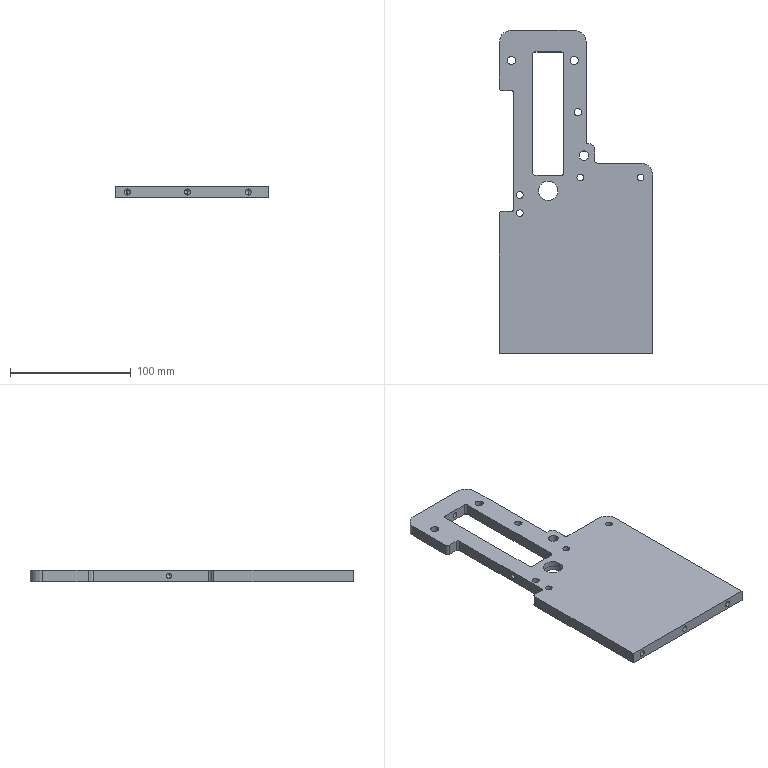Component | SolidWorks | FrameRightPlate.1-1 | 1 solid | 70 faces | box 127 x 268 x 9.4 mm | volume 221340 mm3 | cylinder 43 | plane 19 | cone 8 | commonest cylinder face diameters 4 x9 5.5 x8 5 x6 4.2 x4 6.8 x4 20 x3 16 x2 8 x2
build123d program:
from build123d import *

# Parameters (mm, degrees)
SKETCH1_R                      = 9.5
SKETCH1_R_2                    = 3
SKETCH1_R_3                    = 4
BOSS_EXTRUDE1_DEPTH            = 9.4
M8_TAPPED_HOLE1_D              = 6.8
M8_TAPPED_HOLE1_DEPTH          = 19.75
M8_TAPPED_HOLE1_TIP            = 2.043
F_5_5_5_5_DIAMETER_HOLE1_D     = 5.5
F_5_5_5_5_DIAMETER_HOLE1_DEPTH = 10
F_5_5_5_5_DIAMETER_HOLE1_TIP   = 1.652
F_5_5_5_5_DIAMETER_HOLE2_D     = 5.5
F_5_5_5_5_DIAMETER_HOLE2_DEPTH = 10
F_5_5_5_5_DIAMETER_HOLE2_TIP   = 1.652
M5_TAPPED_HOLE3_D              = 4.2
M5_TAPPED_HOLE3_DEPTH          = 12.4
M5_TAPPED_HOLE3_TIP            = 1.262
M5_TAPPED_HOLE4_D              = 4.2
M5_TAPPED_HOLE4_DEPTH          = 20
M5_TAPPED_HOLE4_TIP            = 1.262
M6_TAPPED_HOLE1_D              = 5
M6_TAPPED_HOLE1_DEPTH          = 15
M6_TAPPED_HOLE1_TIP            = 1.502
BOSS_EXTRUDE2_START            = -5
SKETCH14_R                     = 9.5
SKETCH14_R_2                   = 8
BOSS_EXTRUDE2_DEPTH            = 4.4


with BuildPart() as part:
    # Sketch1 → Boss-Extrude1 (new body)
    with BuildSketch(Plane.XY):
        with BuildLine():
            Line((81, 158), (117, 158))
            ThreePointArc((117, 158), (124.071, 155.071), (127, 148))
            Line((127, 148), (127, 0))
            Line((127, 0), (0, 0))
            Line((0, 0), (0, 116))
            ThreePointArc((0, 116), (0.5858, 117.414), (2, 118))
            Line((2, 118), (10, 118))
            ThreePointArc((10, 118), (11.414, 118.586), (12, 120))
            Line((12, 120), (12, 216))
            ThreePointArc((12, 216), (11.414, 217.414), (10, 218))
            Line((10, 218), (2, 218))
            ThreePointArc((2, 218), (0.5858, 218.586), (0, 220))
            Line((0, 220), (0, 258))
            ThreePointArc((0, 258), (2.929, 265.071), (10, 268))
            Line((10, 268), (62, 268))
            ThreePointArc((62, 268), (69.071, 265.071), (72, 258))
            Line((72, 258), (72, 174))
            Line((72, 174), (74, 174))
            ThreePointArc((74, 174), (77.536, 172.536), (79, 169))
            Line((79, 169), (79, 160))
            ThreePointArc((79, 160), (79.586, 158.586), (81, 158))
        make_face()
        with Locations((40.5, 135)):
            Circle(SKETCH1_R, mode=Mode.SUBTRACT)
        with Locations((65, 200)):
            Circle(SKETCH1_R_2, mode=Mode.SUBTRACT)
        with Locations((70, 164)):
            Circle(SKETCH1_R_3, mode=Mode.SUBTRACT)
        with BuildLine():
            Line((29.5, 250), (51.5, 250))
            ThreePointArc((51.5, 250), (52.914, 249.414), (53.5, 248))
            Line((53.5, 248), (53.5, 150))
            ThreePointArc((53.5, 150), (52.914, 148.586), (51.5, 148))
            Line((51.5, 148), (29.5, 148))
            ThreePointArc((29.5, 148), (28.086, 148.586), (27.5, 150))
            Line((27.5, 150), (27.5, 248))
            ThreePointArc((27.5, 248), (28.086, 249.414), (29.5, 250))
        make_face(mode=Mode.SUBTRACT)
    extrude(amount=BOSS_EXTRUDE1_DEPTH)

    # M8 Tapped Hole1
    with Locations(Plane.XY.offset(9.4)):
        with Locations((62, 243), (10, 243)):
            Hole(M8_TAPPED_HOLE1_D / 2, depth=M8_TAPPED_HOLE1_DEPTH)
            with Locations((0, 0, -(M8_TAPPED_HOLE1_DEPTH + M8_TAPPED_HOLE1_TIP / 2))):  # 118° drill point
                Cone(0, M8_TAPPED_HOLE1_D / 2, M8_TAPPED_HOLE1_TIP, mode=Mode.SUBTRACT)

    # 5.5 _5.5_ Diameter Hole1
    with Locations(Plane.XY.offset(9.4)):
        with Locations((17, 131.5), (17, 116.5)):
            Hole(F_5_5_5_5_DIAMETER_HOLE1_D / 2, depth=F_5_5_5_5_DIAMETER_HOLE1_DEPTH)
            with Locations((0, 0, -(F_5_5_5_5_DIAMETER_HOLE1_DEPTH + F_5_5_5_5_DIAMETER_HOLE1_TIP / 2))):  # 118° drill point
                Cone(0, F_5_5_5_5_DIAMETER_HOLE1_D / 2, F_5_5_5_5_DIAMETER_HOLE1_TIP, mode=Mode.SUBTRACT)

    # 5.5 _5.5_ Diameter Hole2
    with Locations(Plane.XY.offset(9.4)):
        with Locations((117, 146), (67, 146)):
            Hole(F_5_5_5_5_DIAMETER_HOLE2_D / 2, depth=F_5_5_5_5_DIAMETER_HOLE2_DEPTH)
            with Locations((0, 0, -(F_5_5_5_5_DIAMETER_HOLE2_DEPTH + F_5_5_5_5_DIAMETER_HOLE2_TIP / 2))):  # 118° drill point
                Cone(0, F_5_5_5_5_DIAMETER_HOLE2_D / 2, F_5_5_5_5_DIAMETER_HOLE2_TIP, mode=Mode.SUBTRACT)

    # M5 Tapped Hole3
    with Locations(Plane.ZY.offset(-12)):
        with Locations((4.9, 153)):
            Hole(M5_TAPPED_HOLE3_D / 2, depth=M5_TAPPED_HOLE3_DEPTH)
            with Locations((0, 0, -(M5_TAPPED_HOLE3_DEPTH + M5_TAPPED_HOLE3_TIP / 2))):  # 118° drill point
                Cone(0, M5_TAPPED_HOLE3_D / 2, M5_TAPPED_HOLE3_TIP, mode=Mode.SUBTRACT)

    # M5 Tapped Hole4
    with Locations(Plane(origin=(0, 268, 0), x_dir=(-1, 0, 0), z_dir=(0, 1, 0))):
        with Locations((-40.5, 4.7)):
            Hole(M5_TAPPED_HOLE4_D / 2, depth=M5_TAPPED_HOLE4_DEPTH)
            with Locations((0, 0, -(M5_TAPPED_HOLE4_DEPTH + M5_TAPPED_HOLE4_TIP / 2))):  # 118° drill point
                Cone(0, M5_TAPPED_HOLE4_D / 2, M5_TAPPED_HOLE4_TIP, mode=Mode.SUBTRACT)

    # M6 Tapped Hole1
    with Locations(Plane.XZ):
        with Locations((10, 4.7), (60, 4.7), (110, 4.7)):
            Hole(M6_TAPPED_HOLE1_D / 2, depth=M6_TAPPED_HOLE1_DEPTH)
            with Locations((0, 0, -(M6_TAPPED_HOLE1_DEPTH + M6_TAPPED_HOLE1_TIP / 2))):  # 118° drill point
                Cone(0, M6_TAPPED_HOLE1_D / 2, M6_TAPPED_HOLE1_TIP, mode=Mode.SUBTRACT)

    # Sketch14 → Boss-Extrude2 (add)
    with BuildSketch(Plane(origin=(0, 0, 0), x_dir=(-1, 0, 0), z_dir=(0, 0, -1)).offset(BOSS_EXTRUDE2_START)):
        with Locations((-40.5, 135)):
            Circle(SKETCH14_R)
        with Locations((-40.5, 135)):
            Circle(SKETCH14_R_2, mode=Mode.SUBTRACT)
    extrude(amount=-BOSS_EXTRUDE2_DEPTH)


solid = part.part

# Placed as in the assembly
solid = solid.moved(Location((0, 0, 70), (0, 0, 0)))